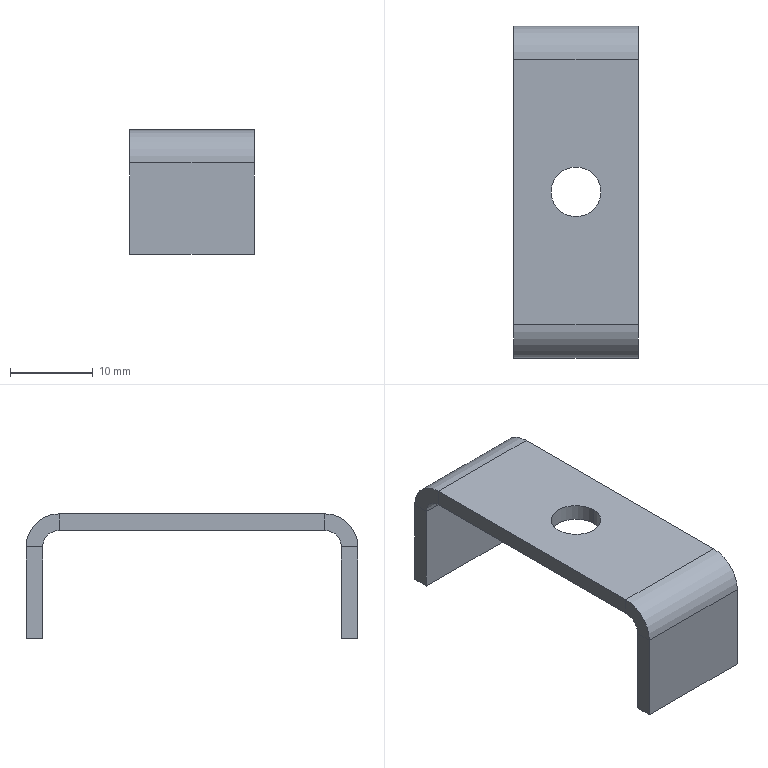Component | SolidWorks | SidePanelAssembly-1_BindingWireRack-14 | 1 solid | 24 faces | box 15 x 40 x 15 mm | volume 1846 mm3 | plane 18 | cylinder 6 | commonest cylinder face diameters 6 x2 8 x2 4 x2
STEP:
#1=COLOUR_RGB('',0.7922,0.8196,0.9333);
#2=FILL_AREA_STYLE_COLOUR('',#1);
#3=FILL_AREA_STYLE('',(#2));
#4=SURFACE_STYLE_FILL_AREA(#3);
#5=SURFACE_SIDE_STYLE('',(#4));
#6=SURFACE_STYLE_USAGE(.BOTH.,#5);
#7=PRESENTATION_STYLE_ASSIGNMENT((#6));
#8=CARTESIAN_POINT('',(26.468,42.957,-22.992));
#9=VERTEX_POINT('',#8);
#10=CARTESIAN_POINT('',(26.232,42.957,-22.992));
#11=VERTEX_POINT('',#10);
#12=CARTESIAN_POINT('',(26.35,42.957,-22.992));
#13=DIRECTION('',(-0.,-0.,1.));
#14=DIRECTION('',(-1.,0.,0.));
#15=AXIS2_PLACEMENT_3D('',#12,#13,#14);
#16=CIRCLE('',#15,0.1181);
#17=EDGE_CURVE('',#9,#11,#16,.T.);
#18=ORIENTED_EDGE('',*,*,#17,.F.);
#19=CARTESIAN_POINT('',(26.468,42.957,-22.913));
#20=VERTEX_POINT('',#19);
#21=CARTESIAN_POINT('',(26.468,42.957,-23.307));
#22=DIRECTION('',(-0.,-0.,1.));
#23=VECTOR('',#22,39.37);
#24=LINE('',#21,#23);
#25=EDGE_CURVE('',#9,#20,#24,.T.);
#26=ORIENTED_EDGE('',*,*,#25,.T.);
#27=CARTESIAN_POINT('',(26.232,42.957,-22.913));
#28=VERTEX_POINT('',#27);
#29=CARTESIAN_POINT('',(26.35,42.957,-22.913));
#30=DIRECTION('',(-0.,-0.,1.));
#31=DIRECTION('',(-1.,0.,0.));
#32=AXIS2_PLACEMENT_3D('',#29,#30,#31);
#33=CIRCLE('',#32,0.1181);
#34=EDGE_CURVE('',#20,#28,#33,.T.);
#35=ORIENTED_EDGE('',*,*,#34,.T.);
#36=CARTESIAN_POINT('',(26.232,42.957,-23.307));
#37=DIRECTION('',(-0.,-0.,1.));
#38=VECTOR('',#37,39.37);
#39=LINE('',#36,#38);
#40=EDGE_CURVE('',#11,#28,#39,.T.);
#41=ORIENTED_EDGE('',*,*,#40,.F.);
#42=EDGE_LOOP('',(#18,#26,#35,#41));
#43=FACE_OUTER_BOUND('',#42,.T.);
#44=CARTESIAN_POINT('',(26.35,42.957,-23.307));
#45=DIRECTION('',(-0.,-0.,1.));
#46=DIRECTION('',(-1.,0.,0.));
#47=AXIS2_PLACEMENT_3D('',#44,#45,#46);
#48=CYLINDRICAL_SURFACE('',#47,0.1181);
#49=ADVANCED_FACE('',(#43),#48,.F.);
#50=CARTESIAN_POINT('',(26.054,43.587,-22.913));
#51=VERTEX_POINT('',#50);
#52=CARTESIAN_POINT('',(26.054,43.587,-22.992));
#53=VERTEX_POINT('',#52);
#54=CARTESIAN_POINT('',(26.054,43.587,-22.913));
#55=DIRECTION('',(0.,0.,-1.));
#56=VECTOR('',#55,39.37);
#57=LINE('',#54,#56);
#58=EDGE_CURVE('',#51,#53,#57,.T.);
#59=ORIENTED_EDGE('',*,*,#58,.F.);
#60=CARTESIAN_POINT('',(26.054,43.744,-23.071));
#61=VERTEX_POINT('',#60);
#62=CARTESIAN_POINT('',(26.054,43.587,-23.071));
#63=DIRECTION('',(1.,-0.,0.));
#64=DIRECTION('',(0.,-1.,0.));
#65=AXIS2_PLACEMENT_3D('',#62,#63,#64);
#66=CIRCLE('',#65,0.1575);
#67=EDGE_CURVE('',#61,#51,#66,.T.);
#68=ORIENTED_EDGE('',*,*,#67,.F.);
#69=CARTESIAN_POINT('',(26.054,43.665,-23.071));
#70=VERTEX_POINT('',#69);
#71=CARTESIAN_POINT('',(26.054,43.665,-23.071));
#72=DIRECTION('',(-0.,1.,0.));
#73=VECTOR('',#72,39.37);
#74=LINE('',#71,#73);
#75=EDGE_CURVE('',#70,#61,#74,.T.);
#76=ORIENTED_EDGE('',*,*,#75,.F.);
#77=CARTESIAN_POINT('',(26.054,43.587,-23.071));
#78=DIRECTION('',(1.,-0.,0.));
#79=DIRECTION('',(0.,-1.,0.));
#80=AXIS2_PLACEMENT_3D('',#77,#78,#79);
#81=CIRCLE('',#80,0.07874);
#82=EDGE_CURVE('',#70,#53,#81,.T.);
#83=ORIENTED_EDGE('',*,*,#82,.T.);
#84=EDGE_LOOP('',(#59,#68,#76,#83));
#85=FACE_OUTER_BOUND('',#84,.T.);
#86=CARTESIAN_POINT('',(26.054,43.587,-22.913));
#87=DIRECTION('',(-1.,-0.,-0.));
#88=DIRECTION('',(0.,-1.,-0.));
#89=AXIS2_PLACEMENT_3D('',#86,#87,#88);
#90=PLANE('',#89);
#91=ADVANCED_FACE('',(#85),#90,.T.);
#92=CARTESIAN_POINT('',(26.054,42.327,-22.913));
#93=VERTEX_POINT('',#92);
#94=CARTESIAN_POINT('',(26.054,43.744,-22.913));
#95=DIRECTION('',(0.,-1.,-0.));
#96=VECTOR('',#95,39.37);
#97=LINE('',#94,#96);
#98=EDGE_CURVE('',#51,#93,#97,.T.);
#99=ORIENTED_EDGE('',*,*,#98,.F.);
#100=ORIENTED_EDGE('',*,*,#58,.T.);
#101=CARTESIAN_POINT('',(26.054,42.327,-22.992));
#102=VERTEX_POINT('',#101);
#103=CARTESIAN_POINT('',(26.054,43.744,-22.992));
#104=DIRECTION('',(0.,-1.,-0.));
#105=VECTOR('',#104,39.37);
#106=LINE('',#103,#105);
#107=EDGE_CURVE('',#53,#102,#106,.T.);
#108=ORIENTED_EDGE('',*,*,#107,.T.);
#109=CARTESIAN_POINT('',(26.054,42.327,-22.992));
#110=DIRECTION('',(-0.,-0.,1.));
#111=VECTOR('',#110,39.37);
#112=LINE('',#109,#111);
#113=EDGE_CURVE('',#102,#93,#112,.T.);
#114=ORIENTED_EDGE('',*,*,#113,.T.);
#115=EDGE_LOOP('',(#99,#100,#108,#114));
#116=FACE_OUTER_BOUND('',#115,.T.);
#117=CARTESIAN_POINT('',(26.054,43.665,-23.071));
#118=DIRECTION('',(-1.,-0.,-0.));
#119=DIRECTION('',(0.,-1.,-0.));
#120=AXIS2_PLACEMENT_3D('',#117,#118,#119);
#121=PLANE('',#120);
#122=ADVANCED_FACE('',(#116),#121,.T.);
#123=CARTESIAN_POINT('',(26.645,43.744,-23.071));
#124=VERTEX_POINT('',#123);
#125=CARTESIAN_POINT('',(26.645,43.665,-23.071));
#126=VERTEX_POINT('',#125);
#127=CARTESIAN_POINT('',(26.645,43.744,-23.071));
#128=DIRECTION('',(0.,-1.,-0.));
#129=VECTOR('',#128,39.37);
#130=LINE('',#127,#129);
#131=EDGE_CURVE('',#124,#126,#130,.T.);
#132=ORIENTED_EDGE('',*,*,#131,.F.);
#133=CARTESIAN_POINT('',(26.645,43.587,-22.913));
#134=VERTEX_POINT('',#133);
#135=CARTESIAN_POINT('',(26.645,43.587,-23.071));
#136=DIRECTION('',(1.,-0.,0.));
#137=DIRECTION('',(0.,-1.,0.));
#138=AXIS2_PLACEMENT_3D('',#135,#136,#137);
#139=CIRCLE('',#138,0.1575);
#140=EDGE_CURVE('',#124,#134,#139,.T.);
#141=ORIENTED_EDGE('',*,*,#140,.T.);
#142=CARTESIAN_POINT('',(26.645,43.587,-22.992));
#143=VERTEX_POINT('',#142);
#144=CARTESIAN_POINT('',(26.645,43.587,-22.992));
#145=DIRECTION('',(-0.,-0.,1.));
#146=VECTOR('',#145,39.37);
#147=LINE('',#144,#146);
#148=EDGE_CURVE('',#143,#134,#147,.T.);
#149=ORIENTED_EDGE('',*,*,#148,.F.);
#150=CARTESIAN_POINT('',(26.645,43.587,-23.071));
#151=DIRECTION('',(1.,-0.,0.));
#152=DIRECTION('',(0.,-1.,0.));
#153=AXIS2_PLACEMENT_3D('',#150,#151,#152);
#154=CIRCLE('',#153,0.07874);
#155=EDGE_CURVE('',#126,#143,#154,.T.);
#156=ORIENTED_EDGE('',*,*,#155,.F.);
#157=EDGE_LOOP('',(#132,#141,#149,#156));
#158=FACE_OUTER_BOUND('',#157,.T.);
#159=CARTESIAN_POINT('',(26.645,43.744,-23.071));
#160=DIRECTION('',(1.,0.,0.));
#161=DIRECTION('',(-0.,1.,0.));
#162=AXIS2_PLACEMENT_3D('',#159,#160,#161);
#163=PLANE('',#162);
#164=ADVANCED_FACE('',(#158),#163,.T.);
#165=CARTESIAN_POINT('',(26.645,43.744,-23.504));
#166=VERTEX_POINT('',#165);
#167=CARTESIAN_POINT('',(26.645,43.744,-23.504));
#168=DIRECTION('',(-0.,-0.,1.));
#169=VECTOR('',#168,39.37);
#170=LINE('',#167,#169);
#171=EDGE_CURVE('',#166,#124,#170,.T.);
#172=ORIENTED_EDGE('',*,*,#171,.T.);
#173=ORIENTED_EDGE('',*,*,#131,.T.);
#174=CARTESIAN_POINT('',(26.645,43.665,-23.504));
#175=VERTEX_POINT('',#174);
#176=CARTESIAN_POINT('',(26.645,43.665,-23.504));
#177=DIRECTION('',(-0.,-0.,1.));
#178=VECTOR('',#177,39.37);
#179=LINE('',#176,#178);
#180=EDGE_CURVE('',#175,#126,#179,.T.);
#181=ORIENTED_EDGE('',*,*,#180,.F.);
#182=CARTESIAN_POINT('',(26.645,43.665,-23.504));
#183=DIRECTION('',(-0.,1.,0.));
#184=VECTOR('',#183,39.37);
#185=LINE('',#182,#184);
#186=EDGE_CURVE('',#175,#166,#185,.T.);
#187=ORIENTED_EDGE('',*,*,#186,.T.);
#188=EDGE_LOOP('',(#172,#173,#181,#187));
#189=FACE_OUTER_BOUND('',#188,.T.);
#190=CARTESIAN_POINT('',(26.645,43.587,-22.992));
#191=DIRECTION('',(1.,0.,0.));
#192=DIRECTION('',(-0.,1.,0.));
#193=AXIS2_PLACEMENT_3D('',#190,#191,#192);
#194=PLANE('',#193);
#195=ADVANCED_FACE('',(#189),#194,.T.);
#196=CARTESIAN_POINT('',(26.054,42.169,-23.071));
#197=VERTEX_POINT('',#196);
#198=CARTESIAN_POINT('',(26.054,42.248,-23.071));
#199=VERTEX_POINT('',#198);
#200=CARTESIAN_POINT('',(26.054,42.169,-23.071));
#201=DIRECTION('',(-0.,1.,0.));
#202=VECTOR('',#201,39.37);
#203=LINE('',#200,#202);
#204=EDGE_CURVE('',#197,#199,#203,.T.);
#205=ORIENTED_EDGE('',*,*,#204,.F.);
#206=CARTESIAN_POINT('',(26.054,42.327,-23.071));
#207=DIRECTION('',(1.,-0.,0.));
#208=DIRECTION('',(0.,-1.,-0.));
#209=AXIS2_PLACEMENT_3D('',#206,#207,#208);
#210=CIRCLE('',#209,0.1575);
#211=EDGE_CURVE('',#93,#197,#210,.T.);
#212=ORIENTED_EDGE('',*,*,#211,.F.);
#213=ORIENTED_EDGE('',*,*,#113,.F.);
#214=CARTESIAN_POINT('',(26.054,42.327,-23.071));
#215=DIRECTION('',(1.,-0.,0.));
#216=DIRECTION('',(0.,-1.,0.));
#217=AXIS2_PLACEMENT_3D('',#214,#215,#216);
#218=CIRCLE('',#217,0.07874);
#219=EDGE_CURVE('',#102,#199,#218,.T.);
#220=ORIENTED_EDGE('',*,*,#219,.T.);
#221=EDGE_LOOP('',(#205,#212,#213,#220));
#222=FACE_OUTER_BOUND('',#221,.T.);
#223=CARTESIAN_POINT('',(26.054,42.169,-23.071));
#224=DIRECTION('',(-1.,-0.,-0.));
#225=DIRECTION('',(0.,-1.,-0.));
#226=AXIS2_PLACEMENT_3D('',#223,#224,#225);
#227=PLANE('',#226);
#228=ADVANCED_FACE('',(#222),#227,.T.);
#229=CARTESIAN_POINT('',(26.054,42.169,-23.504));
#230=VERTEX_POINT('',#229);
#231=CARTESIAN_POINT('',(26.054,42.169,-22.913));
#232=DIRECTION('',(0.,0.,-1.));
#233=VECTOR('',#232,39.37);
#234=LINE('',#231,#233);
#235=EDGE_CURVE('',#197,#230,#234,.T.);
#236=ORIENTED_EDGE('',*,*,#235,.F.);
#237=ORIENTED_EDGE('',*,*,#204,.T.);
#238=CARTESIAN_POINT('',(26.054,42.248,-23.504));
#239=VERTEX_POINT('',#238);
#240=CARTESIAN_POINT('',(26.054,42.248,-22.913));
#241=DIRECTION('',(0.,0.,-1.));
#242=VECTOR('',#241,39.37);
#243=LINE('',#240,#242);
#244=EDGE_CURVE('',#199,#239,#243,.T.);
#245=ORIENTED_EDGE('',*,*,#244,.T.);
#246=CARTESIAN_POINT('',(26.054,42.169,-23.504));
#247=DIRECTION('',(-0.,1.,0.));
#248=VECTOR('',#247,39.37);
#249=LINE('',#246,#248);
#250=EDGE_CURVE('',#230,#239,#249,.T.);
#251=ORIENTED_EDGE('',*,*,#250,.F.);
#252=EDGE_LOOP('',(#236,#237,#245,#251));
#253=FACE_OUTER_BOUND('',#252,.T.);
#254=CARTESIAN_POINT('',(26.054,42.327,-22.992));
#255=DIRECTION('',(-1.,-0.,-0.));
#256=DIRECTION('',(0.,-1.,-0.));
#257=AXIS2_PLACEMENT_3D('',#254,#255,#256);
#258=PLANE('',#257);
#259=ADVANCED_FACE('',(#253),#258,.T.);
#260=CARTESIAN_POINT('',(26.645,42.327,-22.913));
#261=VERTEX_POINT('',#260);
#262=CARTESIAN_POINT('',(26.645,42.327,-22.992));
#263=VERTEX_POINT('',#262);
#264=CARTESIAN_POINT('',(26.645,42.327,-22.913));
#265=DIRECTION('',(0.,0.,-1.));
#266=VECTOR('',#265,39.37);
#267=LINE('',#264,#266);
#268=EDGE_CURVE('',#261,#263,#267,.T.);
#269=ORIENTED_EDGE('',*,*,#268,.F.);
#270=CARTESIAN_POINT('',(26.645,42.169,-23.071));
#271=VERTEX_POINT('',#270);
#272=CARTESIAN_POINT('',(26.645,42.327,-23.071));
#273=DIRECTION('',(1.,-0.,0.));
#274=DIRECTION('',(0.,-1.,-0.));
#275=AXIS2_PLACEMENT_3D('',#272,#273,#274);
#276=CIRCLE('',#275,0.1575);
#277=EDGE_CURVE('',#261,#271,#276,.T.);
#278=ORIENTED_EDGE('',*,*,#277,.T.);
#279=CARTESIAN_POINT('',(26.645,42.248,-23.071));
#280=VERTEX_POINT('',#279);
#281=CARTESIAN_POINT('',(26.645,42.248,-23.071));
#282=DIRECTION('',(0.,-1.,-0.));
#283=VECTOR('',#282,39.37);
#284=LINE('',#281,#283);
#285=EDGE_CURVE('',#280,#271,#284,.T.);
#286=ORIENTED_EDGE('',*,*,#285,.F.);
#287=CARTESIAN_POINT('',(26.645,42.327,-23.071));
#288=DIRECTION('',(1.,-0.,0.));
#289=DIRECTION('',(0.,-1.,0.));
#290=AXIS2_PLACEMENT_3D('',#287,#288,#289);
#291=CIRCLE('',#290,0.07874);
#292=EDGE_CURVE('',#263,#280,#291,.T.);
#293=ORIENTED_EDGE('',*,*,#292,.F.);
#294=EDGE_LOOP('',(#269,#278,#286,#293));
#295=FACE_OUTER_BOUND('',#294,.T.);
#296=CARTESIAN_POINT('',(26.645,42.327,-22.913));
#297=DIRECTION('',(1.,0.,0.));
#298=DIRECTION('',(-0.,1.,0.));
#299=AXIS2_PLACEMENT_3D('',#296,#297,#298);
#300=PLANE('',#299);
#301=ADVANCED_FACE('',(#295),#300,.T.);
#302=CARTESIAN_POINT('',(26.645,43.744,-22.913));
#303=DIRECTION('',(0.,-1.,-0.));
#304=VECTOR('',#303,39.37);
#305=LINE('',#302,#304);
#306=EDGE_CURVE('',#134,#261,#305,.T.);
#307=ORIENTED_EDGE('',*,*,#306,.T.);
#308=ORIENTED_EDGE('',*,*,#268,.T.);
#309=CARTESIAN_POINT('',(26.645,43.744,-22.992));
#310=DIRECTION('',(0.,-1.,-0.));
#311=VECTOR('',#310,39.37);
#312=LINE('',#309,#311);
#313=EDGE_CURVE('',#143,#263,#312,.T.);
#314=ORIENTED_EDGE('',*,*,#313,.F.);
#315=ORIENTED_EDGE('',*,*,#148,.T.);
#316=EDGE_LOOP('',(#307,#308,#314,#315));
#317=FACE_OUTER_BOUND('',#316,.T.);
#318=CARTESIAN_POINT('',(26.645,42.248,-23.071));
#319=DIRECTION('',(1.,0.,0.));
#320=DIRECTION('',(-0.,1.,0.));
#321=AXIS2_PLACEMENT_3D('',#318,#319,#320);
#322=PLANE('',#321);
#323=ADVANCED_FACE('',(#317),#322,.T.);
#324=CARTESIAN_POINT('',(26.645,42.248,-23.504));
#325=VERTEX_POINT('',#324);
#326=CARTESIAN_POINT('',(26.645,42.248,-22.913));
#327=DIRECTION('',(0.,0.,-1.));
#328=VECTOR('',#327,39.37);
#329=LINE('',#326,#328);
#330=EDGE_CURVE('',#280,#325,#329,.T.);
#331=ORIENTED_EDGE('',*,*,#330,.T.);
#332=CARTESIAN_POINT('',(26.054,42.248,-23.504));
#333=DIRECTION('',(1.,-0.,0.));
#334=VECTOR('',#333,39.37);
#335=LINE('',#332,#334);
#336=EDGE_CURVE('',#239,#325,#335,.T.);
#337=ORIENTED_EDGE('',*,*,#336,.F.);
#338=ORIENTED_EDGE('',*,*,#244,.F.);
#339=CARTESIAN_POINT('',(26.054,42.248,-23.071));
#340=DIRECTION('',(1.,-0.,0.));
#341=VECTOR('',#340,39.37);
#342=LINE('',#339,#341);
#343=EDGE_CURVE('',#199,#280,#342,.T.);
#344=ORIENTED_EDGE('',*,*,#343,.T.);
#345=EDGE_LOOP('',(#331,#337,#338,#344));
#346=FACE_OUTER_BOUND('',#345,.T.);
#347=CARTESIAN_POINT('',(26.054,42.248,-22.913));
#348=DIRECTION('',(0.,-1.,-0.));
#349=DIRECTION('',(-0.,-0.,1.));
#350=AXIS2_PLACEMENT_3D('',#347,#348,#349);
#351=PLANE('',#350);
#352=ADVANCED_FACE('',(#346),#351,.F.);
#353=CARTESIAN_POINT('',(26.645,42.169,-23.504));
#354=VERTEX_POINT('',#353);
#355=CARTESIAN_POINT('',(26.645,42.169,-23.504));
#356=DIRECTION('',(-0.,1.,0.));
#357=VECTOR('',#356,39.37);
#358=LINE('',#355,#357);
#359=EDGE_CURVE('',#354,#325,#358,.T.);
#360=ORIENTED_EDGE('',*,*,#359,.F.);
#361=CARTESIAN_POINT('',(26.054,42.169,-23.504));
#362=DIRECTION('',(1.,-0.,0.));
#363=VECTOR('',#362,39.37);
#364=LINE('',#361,#363);
#365=EDGE_CURVE('',#230,#354,#364,.T.);
#366=ORIENTED_EDGE('',*,*,#365,.F.);
#367=ORIENTED_EDGE('',*,*,#250,.T.);
#368=ORIENTED_EDGE('',*,*,#336,.T.);
#369=EDGE_LOOP('',(#360,#366,#367,#368));
#370=FACE_OUTER_BOUND('',#369,.T.);
#371=CARTESIAN_POINT('',(26.054,42.169,-23.504));
#372=DIRECTION('',(0.,0.,-1.));
#373=DIRECTION('',(0.,-1.,-0.));
#374=AXIS2_PLACEMENT_3D('',#371,#372,#373);
#375=PLANE('',#374);
#376=ADVANCED_FACE('',(#370),#375,.T.);
#377=CARTESIAN_POINT('',(26.645,42.169,-22.913));
#378=DIRECTION('',(0.,0.,-1.));
#379=VECTOR('',#378,39.37);
#380=LINE('',#377,#379);
#381=EDGE_CURVE('',#271,#354,#380,.T.);
#382=ORIENTED_EDGE('',*,*,#381,.F.);
#383=CARTESIAN_POINT('',(26.054,42.169,-23.071));
#384=DIRECTION('',(1.,-0.,0.));
#385=VECTOR('',#384,39.37);
#386=LINE('',#383,#385);
#387=EDGE_CURVE('',#197,#271,#386,.T.);
#388=ORIENTED_EDGE('',*,*,#387,.F.);
#389=ORIENTED_EDGE('',*,*,#235,.T.);
#390=ORIENTED_EDGE('',*,*,#365,.T.);
#391=EDGE_LOOP('',(#382,#388,#389,#390));
#392=FACE_OUTER_BOUND('',#391,.T.);
#393=CARTESIAN_POINT('',(26.054,42.169,-22.913));
#394=DIRECTION('',(0.,-1.,-0.));
#395=DIRECTION('',(-0.,-0.,1.));
#396=AXIS2_PLACEMENT_3D('',#393,#394,#395);
#397=PLANE('',#396);
#398=ADVANCED_FACE('',(#392),#397,.T.);
#399=ORIENTED_EDGE('',*,*,#277,.F.);
#400=CARTESIAN_POINT('',(26.054,42.327,-22.913));
#401=DIRECTION('',(1.,-0.,0.));
#402=VECTOR('',#401,39.37);
#403=LINE('',#400,#402);
#404=EDGE_CURVE('',#93,#261,#403,.T.);
#405=ORIENTED_EDGE('',*,*,#404,.F.);
#406=ORIENTED_EDGE('',*,*,#211,.T.);
#407=ORIENTED_EDGE('',*,*,#387,.T.);
#408=EDGE_LOOP('',(#399,#405,#406,#407));
#409=FACE_OUTER_BOUND('',#408,.T.);
#410=CARTESIAN_POINT('',(26.054,42.327,-23.071));
#411=DIRECTION('',(1.,-0.,0.));
#412=DIRECTION('',(0.,1.,0.));
#413=AXIS2_PLACEMENT_3D('',#410,#411,#412);
#414=CYLINDRICAL_SURFACE('',#413,0.1575);
#415=ADVANCED_FACE('',(#409),#414,.T.);
#416=CARTESIAN_POINT('',(26.35,42.957,-22.913));
#417=DIRECTION('',(-0.,-0.,1.));
#418=DIRECTION('',(-1.,0.,0.));
#419=AXIS2_PLACEMENT_3D('',#416,#417,#418);
#420=CIRCLE('',#419,0.1181);
#421=EDGE_CURVE('',#28,#20,#420,.T.);
#422=ORIENTED_EDGE('',*,*,#421,.F.);
#423=ORIENTED_EDGE('',*,*,#34,.F.);
#424=EDGE_LOOP('',(#422,#423));
#425=FACE_BOUND('',#424,.T.);
#426=ORIENTED_EDGE('',*,*,#306,.F.);
#427=CARTESIAN_POINT('',(26.054,43.587,-22.913));
#428=DIRECTION('',(1.,-0.,0.));
#429=VECTOR('',#428,39.37);
#430=LINE('',#427,#429);
#431=EDGE_CURVE('',#51,#134,#430,.T.);
#432=ORIENTED_EDGE('',*,*,#431,.F.);
#433=ORIENTED_EDGE('',*,*,#98,.T.);
#434=ORIENTED_EDGE('',*,*,#404,.T.);
#435=EDGE_LOOP('',(#426,#432,#433,#434));
#436=FACE_OUTER_BOUND('',#435,.T.);
#437=CARTESIAN_POINT('',(26.054,43.744,-22.913));
#438=DIRECTION('',(-0.,-0.,1.));
#439=DIRECTION('',(-1.,0.,-0.));
#440=AXIS2_PLACEMENT_3D('',#437,#438,#439);
#441=PLANE('',#440);
#442=ADVANCED_FACE('',(#425,#436),#441,.T.);
#443=ORIENTED_EDGE('',*,*,#140,.F.);
#444=CARTESIAN_POINT('',(26.054,43.744,-23.071));
#445=DIRECTION('',(1.,-0.,0.));
#446=VECTOR('',#445,39.37);
#447=LINE('',#444,#446);
#448=EDGE_CURVE('',#61,#124,#447,.T.);
#449=ORIENTED_EDGE('',*,*,#448,.F.);
#450=ORIENTED_EDGE('',*,*,#67,.T.);
#451=ORIENTED_EDGE('',*,*,#431,.T.);
#452=EDGE_LOOP('',(#443,#449,#450,#451));
#453=FACE_OUTER_BOUND('',#452,.T.);
#454=CARTESIAN_POINT('',(26.054,43.587,-23.071));
#455=DIRECTION('',(1.,-0.,0.));
#456=DIRECTION('',(0.,1.,0.));
#457=AXIS2_PLACEMENT_3D('',#454,#455,#456);
#458=CYLINDRICAL_SURFACE('',#457,0.1575);
#459=ADVANCED_FACE('',(#453),#458,.T.);
#460=ORIENTED_EDGE('',*,*,#171,.F.);
#461=CARTESIAN_POINT('',(26.054,43.744,-23.504));
#462=VERTEX_POINT('',#461);
#463=CARTESIAN_POINT('',(26.054,43.744,-23.504));
#464=DIRECTION('',(1.,-0.,0.));
#465=VECTOR('',#464,39.37);
#466=LINE('',#463,#465);
#467=EDGE_CURVE('',#462,#166,#466,.T.);
#468=ORIENTED_EDGE('',*,*,#467,.F.);
#469=CARTESIAN_POINT('',(26.054,43.744,-23.504));
#470=DIRECTION('',(-0.,-0.,1.));
#471=VECTOR('',#470,39.37);
#472=LINE('',#469,#471);
#473=EDGE_CURVE('',#462,#61,#472,.T.);
#474=ORIENTED_EDGE('',*,*,#473,.T.);
#475=ORIENTED_EDGE('',*,*,#448,.T.);
#476=EDGE_LOOP('',(#460,#468,#474,#475));
#477=FACE_OUTER_BOUND('',#476,.T.);
#478=CARTESIAN_POINT('',(26.054,43.744,-23.504));
#479=DIRECTION('',(0.,1.,0.));
#480=DIRECTION('',(-1.,0.,-0.));
#481=AXIS2_PLACEMENT_3D('',#478,#479,#480);
#482=PLANE('',#481);
#483=ADVANCED_FACE('',(#477),#482,.T.);
#484=ORIENTED_EDGE('',*,*,#186,.F.);
#485=CARTESIAN_POINT('',(26.054,43.665,-23.504));
#486=VERTEX_POINT('',#485);
#487=CARTESIAN_POINT('',(26.054,43.665,-23.504));
#488=DIRECTION('',(1.,-0.,0.));
#489=VECTOR('',#488,39.37);
#490=LINE('',#487,#489);
#491=EDGE_CURVE('',#486,#175,#490,.T.);
#492=ORIENTED_EDGE('',*,*,#491,.F.);
#493=CARTESIAN_POINT('',(26.054,43.665,-23.504));
#494=DIRECTION('',(-0.,1.,0.));
#495=VECTOR('',#494,39.37);
#496=LINE('',#493,#495);
#497=EDGE_CURVE('',#486,#462,#496,.T.);
#498=ORIENTED_EDGE('',*,*,#497,.T.);
#499=ORIENTED_EDGE('',*,*,#467,.T.);
#500=EDGE_LOOP('',(#484,#492,#498,#499));
#501=FACE_OUTER_BOUND('',#500,.T.);
#502=CARTESIAN_POINT('',(26.054,43.665,-23.504));
#503=DIRECTION('',(0.,0.,-1.));
#504=DIRECTION('',(1.,-0.,0.));
#505=AXIS2_PLACEMENT_3D('',#502,#503,#504);
#506=PLANE('',#505);
#507=ADVANCED_FACE('',(#501),#506,.T.);
#508=ORIENTED_EDGE('',*,*,#180,.T.);
#509=CARTESIAN_POINT('',(26.054,43.665,-23.071));
#510=DIRECTION('',(1.,-0.,0.));
#511=VECTOR('',#510,39.37);
#512=LINE('',#509,#511);
#513=EDGE_CURVE('',#70,#126,#512,.T.);
#514=ORIENTED_EDGE('',*,*,#513,.F.);
#515=CARTESIAN_POINT('',(26.054,43.665,-23.504));
#516=DIRECTION('',(-0.,-0.,1.));
#517=VECTOR('',#516,39.37);
#518=LINE('',#515,#517);
#519=EDGE_CURVE('',#486,#70,#518,.T.);
#520=ORIENTED_EDGE('',*,*,#519,.F.);
#521=ORIENTED_EDGE('',*,*,#491,.T.);
#522=EDGE_LOOP('',(#508,#514,#520,#521));
#523=FACE_OUTER_BOUND('',#522,.T.);
#524=CARTESIAN_POINT('',(26.054,43.665,-23.504));
#525=DIRECTION('',(0.,1.,0.));
#526=DIRECTION('',(-1.,0.,-0.));
#527=AXIS2_PLACEMENT_3D('',#524,#525,#526);
#528=PLANE('',#527);
#529=ADVANCED_FACE('',(#523),#528,.F.);
#530=ORIENTED_EDGE('',*,*,#155,.T.);
#531=CARTESIAN_POINT('',(26.054,43.587,-22.992));
#532=DIRECTION('',(1.,-0.,0.));
#533=VECTOR('',#532,39.37);
#534=LINE('',#531,#533);
#535=EDGE_CURVE('',#53,#143,#534,.T.);
#536=ORIENTED_EDGE('',*,*,#535,.F.);
#537=ORIENTED_EDGE('',*,*,#82,.F.);
#538=ORIENTED_EDGE('',*,*,#513,.T.);
#539=EDGE_LOOP('',(#530,#536,#537,#538));
#540=FACE_OUTER_BOUND('',#539,.T.);
#541=CARTESIAN_POINT('',(26.054,43.587,-23.071));
#542=DIRECTION('',(1.,-0.,0.));
#543=DIRECTION('',(0.,1.,0.));
#544=AXIS2_PLACEMENT_3D('',#541,#542,#543);
#545=CYLINDRICAL_SURFACE('',#544,0.07874);
#546=ADVANCED_FACE('',(#540),#545,.F.);
#547=CARTESIAN_POINT('',(26.35,42.957,-22.992));
#548=DIRECTION('',(-0.,-0.,1.));
#549=DIRECTION('',(-1.,0.,0.));
#550=AXIS2_PLACEMENT_3D('',#547,#548,#549);
#551=CIRCLE('',#550,0.1181);
#552=EDGE_CURVE('',#11,#9,#551,.T.);
#553=ORIENTED_EDGE('',*,*,#552,.T.);
#554=ORIENTED_EDGE('',*,*,#17,.T.);
#555=EDGE_LOOP('',(#553,#554));
#556=FACE_BOUND('',#555,.T.);
#557=ORIENTED_EDGE('',*,*,#313,.T.);
#558=CARTESIAN_POINT('',(26.054,42.327,-22.992));
#559=DIRECTION('',(1.,-0.,0.));
#560=VECTOR('',#559,39.37);
#561=LINE('',#558,#560);
#562=EDGE_CURVE('',#102,#263,#561,.T.);
#563=ORIENTED_EDGE('',*,*,#562,.F.);
#564=ORIENTED_EDGE('',*,*,#107,.F.);
#565=ORIENTED_EDGE('',*,*,#535,.T.);
#566=EDGE_LOOP('',(#557,#563,#564,#565));
#567=FACE_OUTER_BOUND('',#566,.T.);
#568=CARTESIAN_POINT('',(26.054,43.744,-22.992));
#569=DIRECTION('',(-0.,-0.,1.));
#570=DIRECTION('',(-1.,0.,-0.));
#571=AXIS2_PLACEMENT_3D('',#568,#569,#570);
#572=PLANE('',#571);
#573=ADVANCED_FACE('',(#556,#567),#572,.F.);
#574=ORIENTED_EDGE('',*,*,#292,.T.);
#575=ORIENTED_EDGE('',*,*,#343,.F.);
#576=ORIENTED_EDGE('',*,*,#219,.F.);
#577=ORIENTED_EDGE('',*,*,#562,.T.);
#578=EDGE_LOOP('',(#574,#575,#576,#577));
#579=FACE_OUTER_BOUND('',#578,.T.);
#580=CARTESIAN_POINT('',(26.054,42.327,-23.071));
#581=DIRECTION('',(1.,-0.,0.));
#582=DIRECTION('',(0.,1.,0.));
#583=AXIS2_PLACEMENT_3D('',#580,#581,#582);
#584=CYLINDRICAL_SURFACE('',#583,0.07874);
#585=ADVANCED_FACE('',(#579),#584,.F.);
#586=ORIENTED_EDGE('',*,*,#519,.T.);
#587=ORIENTED_EDGE('',*,*,#75,.T.);
#588=ORIENTED_EDGE('',*,*,#473,.F.);
#589=ORIENTED_EDGE('',*,*,#497,.F.);
#590=EDGE_LOOP('',(#586,#587,#588,#589));
#591=FACE_OUTER_BOUND('',#590,.T.);
#592=CARTESIAN_POINT('',(26.054,42.327,-23.071));
#593=DIRECTION('',(-1.,-0.,-0.));
#594=DIRECTION('',(0.,-1.,-0.));
#595=AXIS2_PLACEMENT_3D('',#592,#593,#594);
#596=PLANE('',#595);
#597=ADVANCED_FACE('',(#591),#596,.T.);
#598=ORIENTED_EDGE('',*,*,#330,.F.);
#599=ORIENTED_EDGE('',*,*,#285,.T.);
#600=ORIENTED_EDGE('',*,*,#381,.T.);
#601=ORIENTED_EDGE('',*,*,#359,.T.);
#602=EDGE_LOOP('',(#598,#599,#600,#601));
#603=FACE_OUTER_BOUND('',#602,.T.);
#604=CARTESIAN_POINT('',(26.645,42.327,-23.071));
#605=DIRECTION('',(-1.,-0.,-0.));
#606=DIRECTION('',(0.,-1.,-0.));
#607=AXIS2_PLACEMENT_3D('',#604,#605,#606);
#608=PLANE('',#607);
#609=ADVANCED_FACE('',(#603),#608,.F.);
#610=ORIENTED_EDGE('',*,*,#25,.F.);
#611=ORIENTED_EDGE('',*,*,#552,.F.);
#612=ORIENTED_EDGE('',*,*,#40,.T.);
#613=ORIENTED_EDGE('',*,*,#421,.T.);
#614=EDGE_LOOP('',(#610,#611,#612,#613));
#615=FACE_OUTER_BOUND('',#614,.T.);
#616=CARTESIAN_POINT('',(26.35,42.957,-23.307));
#617=DIRECTION('',(-0.,-0.,1.));
#618=DIRECTION('',(-1.,0.,0.));
#619=AXIS2_PLACEMENT_3D('',#616,#617,#618);
#620=CYLINDRICAL_SURFACE('',#619,0.1181);
#621=ADVANCED_FACE('',(#615),#620,.F.);
#622=CLOSED_SHELL('',(#49,#91,#122,#164,#195,#228,#259,#301,#323,#352,#376,#398,#415,#442,#459,#483,#507,#529,#546,#573,#585,#597,#609,#621));
#623=MANIFOLD_SOLID_BREP('',#622);
#624=STYLED_ITEM('',(#7),#623);
#625=(LENGTH_UNIT()NAMED_UNIT(*)SI_UNIT($,.METRE.));
#626=LENGTH_MEASURE_WITH_UNIT(LENGTH_MEASURE(0.0254),#625);
#627=DIMENSIONAL_EXPONENTS(1.,0.,0.,0.,0.,0.,0.);
#628=(CONVERSION_BASED_UNIT('',#626)LENGTH_UNIT()NAMED_UNIT(#627));
#629=UNCERTAINTY_MEASURE_WITH_UNIT(LENGTH_MEASURE(0.00001),#628,'','');
#630=(NAMED_UNIT(*)PLANE_ANGLE_UNIT()SI_UNIT($,.RADIAN.));
#631=(NAMED_UNIT(*)SI_UNIT($,.STERADIAN.)SOLID_ANGLE_UNIT());
#632=(GEOMETRIC_REPRESENTATION_CONTEXT(3)GLOBAL_UNCERTAINTY_ASSIGNED_CONTEXT((#629))GLOBAL_UNIT_ASSIGNED_CONTEXT((#628,#630,#631))REPRESENTATION_CONTEXT('',''));
#633=MECHANICAL_DESIGN_GEOMETRIC_PRESENTATION_REPRESENTATION('',(#624),#632);
#634=PRESENTATION_LAYER_ASSIGNMENT('','',(#624));
#635=CARTESIAN_POINT('',(0.,0.,0.));
#636=DIRECTION('',(0.,0.,1.));
#637=DIRECTION('',(1.,0.,0.));
#638=AXIS2_PLACEMENT_3D('',#635,#636,#637);
#639=(LENGTH_UNIT()NAMED_UNIT(*)SI_UNIT($,.METRE.));
#640=LENGTH_MEASURE_WITH_UNIT(LENGTH_MEASURE(0.0254),#639);
#641=DIMENSIONAL_EXPONENTS(1.,0.,0.,0.,0.,0.,0.);
#642=(CONVERSION_BASED_UNIT('',#640)LENGTH_UNIT()NAMED_UNIT(#641));
#643=UNCERTAINTY_MEASURE_WITH_UNIT(LENGTH_MEASURE(0.00001),#642,'','');
#644=(NAMED_UNIT(*)PLANE_ANGLE_UNIT()SI_UNIT($,.RADIAN.));
#645=(NAMED_UNIT(*)SI_UNIT($,.STERADIAN.)SOLID_ANGLE_UNIT());
#646=(GEOMETRIC_REPRESENTATION_CONTEXT(3)GLOBAL_UNCERTAINTY_ASSIGNED_CONTEXT((#643))GLOBAL_UNIT_ASSIGNED_CONTEXT((#642,#644,#645))REPRESENTATION_CONTEXT('',''));
#647=ADVANCED_BREP_SHAPE_REPRESENTATION('',(#623,#638),#646);